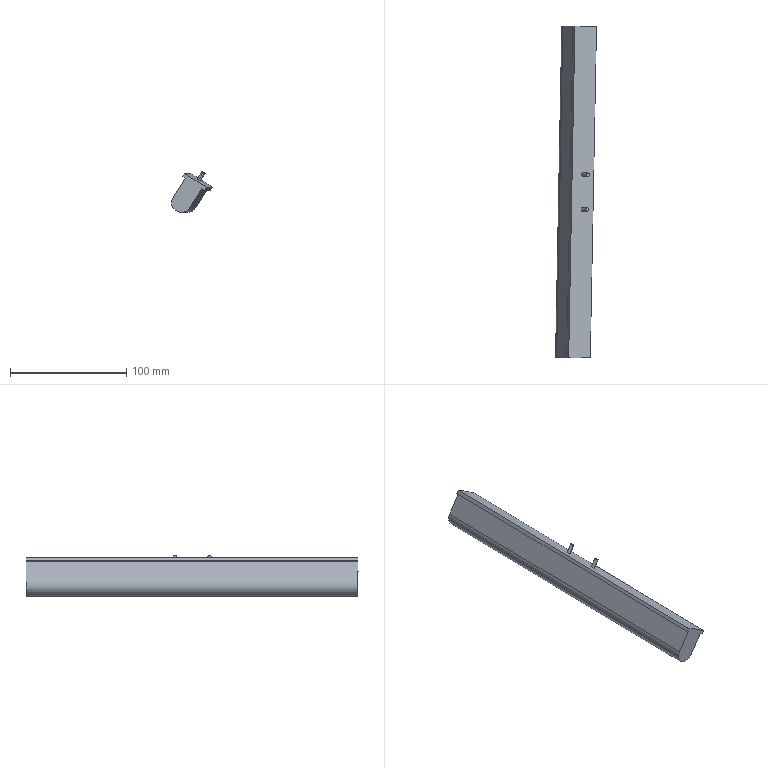Component | SolidWorks | LowerCameraLightSource-1 | 1 solid | 16 faces | box 35.21 x 285.51 x 35.02 mm | volume 145745 mm3 | plane 11 | cylinder 5 | commonest cylinder face diameters 3 x4 17 x1 | material PP Copolymer
build123d program:
from build123d import *

# Parameters (mm, degrees)
BOSS_EXTRUDE1_DEPTH = 142.5
SKETCH2_R           = 1.5
BOSS_EXTRUDE2_DEPTH = 8


with BuildPart() as part:
    # Sketch1 → Boss-Extrude1 (new, symmetric)
    with BuildSketch(Plane.XY):
        with BuildLine():
            Line((-8.5, 0), (-8.5, -19.5))
            Line((-8.5, -19.5), (-11, -19.5))
            Line((-11, -19.5), (-11, -22.5))
            Line((-11, -22.5), (11, -22.5))
            Line((11, -22.5), (11, -19.5))
            Line((11, -19.5), (8.5, -19.5))
            Line((8.5, -19.5), (8.5, 0))
            ThreePointArc((8.5, 0), (0, 8.5), (-8.5, 0))
        make_face()
    extrude(amount=BOSS_EXTRUDE1_DEPTH, both=True)

    # Sketch2 → Boss-Extrude2 (add)
    with BuildSketch(Plane.XZ.offset(22.5)):
        with Locations(Location((0, -15, 0), (0, 0, 90))):
            Circle(SKETCH2_R)
        with Locations(Location((0, 15, 0), (0, 0, 90))):
            Circle(SKETCH2_R)
    extrude(amount=BOSS_EXTRUDE2_DEPTH)


solid = part.part

# Placed as in the assembly
solid = solid.moved(Location((590.931, 385.027, 902.845), (90, -1.073, 147.47)))
STEP:
#1=CARTESIAN_POINT('',(23.901,14.615,36.557));
#2=VERTEX_POINT('',#1);
#3=CARTESIAN_POINT('',(23.898,14.497,36.557));
#4=VERTEX_POINT('',#3);
#5=CARTESIAN_POINT('',(23.9,14.556,36.557));
#6=DIRECTION('',(0.5377,-0.01007,0.8431));
#7=DIRECTION('',(-0.01873,-0.9998,0.));
#8=AXIS2_PLACEMENT_3D('',#5,#6,#7);
#9=CIRCLE('',#8,0.05906);
#10=EDGE_CURVE('',#2,#4,#9,.T.);
#11=ORIENTED_EDGE('',*,*,#10,.F.);
#12=CARTESIAN_POINT('',(23.731,14.618,36.292));
#13=VERTEX_POINT('',#12);
#14=CARTESIAN_POINT('',(23.901,14.615,36.557));
#15=DIRECTION('',(-0.5377,0.01007,-0.8431));
#16=VECTOR('',#15,39.37);
#17=LINE('',#14,#16);
#18=EDGE_CURVE('',#2,#13,#17,.T.);
#19=ORIENTED_EDGE('',*,*,#18,.T.);
#20=CARTESIAN_POINT('',(23.729,14.5,36.292));
#21=VERTEX_POINT('',#20);
#22=CARTESIAN_POINT('',(23.73,14.559,36.292));
#23=DIRECTION('',(0.5377,-0.01007,0.8431));
#24=DIRECTION('',(-0.01873,-0.9998,0.));
#25=AXIS2_PLACEMENT_3D('',#22,#23,#24);
#26=CIRCLE('',#25,0.05906);
#27=EDGE_CURVE('',#13,#21,#26,.T.);
#28=ORIENTED_EDGE('',*,*,#27,.T.);
#29=CARTESIAN_POINT('',(23.898,14.497,36.557));
#30=DIRECTION('',(-0.5377,0.01007,-0.8431));
#31=VECTOR('',#30,39.37);
#32=LINE('',#29,#31);
#33=EDGE_CURVE('',#4,#21,#32,.T.);
#34=ORIENTED_EDGE('',*,*,#33,.F.);
#35=EDGE_LOOP('',(#11,#19,#28,#34));
#36=FACE_OUTER_BOUND('',#35,.T.);
#37=CARTESIAN_POINT('',(23.9,14.556,36.557));
#38=DIRECTION('',(-0.5377,0.01007,-0.8431));
#39=DIRECTION('',(-0.01873,-0.9998,0.));
#40=AXIS2_PLACEMENT_3D('',#37,#38,#39);
#41=CYLINDRICAL_SURFACE('',#40,0.05906);
#42=ADVANCED_FACE('',(#36),#41,.T.);
#43=CARTESIAN_POINT('',(23.923,15.796,36.557));
#44=VERTEX_POINT('',#43);
#45=CARTESIAN_POINT('',(23.921,15.678,36.557));
#46=VERTEX_POINT('',#45);
#47=CARTESIAN_POINT('',(23.922,15.737,36.557));
#48=DIRECTION('',(0.5377,-0.01007,0.8431));
#49=DIRECTION('',(0.01873,0.9998,0.));
#50=AXIS2_PLACEMENT_3D('',#47,#48,#49);
#51=CIRCLE('',#50,0.05906);
#52=EDGE_CURVE('',#44,#46,#51,.T.);
#53=ORIENTED_EDGE('',*,*,#52,.F.);
#54=CARTESIAN_POINT('',(23.753,15.799,36.292));
#55=VERTEX_POINT('',#54);
#56=CARTESIAN_POINT('',(23.923,15.796,36.557));
#57=DIRECTION('',(-0.5377,0.01007,-0.8431));
#58=VECTOR('',#57,39.37);
#59=LINE('',#56,#58);
#60=EDGE_CURVE('',#44,#55,#59,.T.);
#61=ORIENTED_EDGE('',*,*,#60,.T.);
#62=CARTESIAN_POINT('',(23.751,15.681,36.292));
#63=VERTEX_POINT('',#62);
#64=CARTESIAN_POINT('',(23.752,15.74,36.292));
#65=DIRECTION('',(0.5377,-0.01007,0.8431));
#66=DIRECTION('',(-0.01873,-0.9998,0.));
#67=AXIS2_PLACEMENT_3D('',#64,#65,#66);
#68=CIRCLE('',#67,0.05906);
#69=EDGE_CURVE('',#55,#63,#68,.T.);
#70=ORIENTED_EDGE('',*,*,#69,.T.);
#71=CARTESIAN_POINT('',(23.921,15.678,36.557));
#72=DIRECTION('',(-0.5377,0.01007,-0.8431));
#73=VECTOR('',#72,39.37);
#74=LINE('',#71,#73);
#75=EDGE_CURVE('',#46,#63,#74,.T.);
#76=ORIENTED_EDGE('',*,*,#75,.F.);
#77=EDGE_LOOP('',(#53,#61,#70,#76));
#78=FACE_OUTER_BOUND('',#77,.T.);
#79=CARTESIAN_POINT('',(23.922,15.737,36.557));
#80=DIRECTION('',(-0.5377,0.01007,-0.8431));
#81=DIRECTION('',(-0.01873,-0.9998,0.));
#82=AXIS2_PLACEMENT_3D('',#79,#80,#81);
#83=CYLINDRICAL_SURFACE('',#82,0.05906);
#84=ADVANCED_FACE('',(#78),#83,.T.);
#85=CARTESIAN_POINT('',(23.088,20.773,35.725));
#86=VERTEX_POINT('',#85);
#87=CARTESIAN_POINT('',(23.652,20.763,35.365));
#88=VERTEX_POINT('',#87);
#89=CARTESIAN_POINT('',(23.37,20.768,35.545));
#90=DIRECTION('',(-0.01873,-0.9998,0.));
#91=DIRECTION('',(-0.843,0.01579,0.5377));
#92=AXIS2_PLACEMENT_3D('',#89,#90,#91);
#93=CIRCLE('',#92,0.3346);
#94=EDGE_CURVE('',#86,#88,#93,.T.);
#95=ORIENTED_EDGE('',*,*,#94,.T.);
#96=CARTESIAN_POINT('',(23.442,9.544,35.365));
#97=VERTEX_POINT('',#96);
#98=CARTESIAN_POINT('',(23.442,9.544,35.365));
#99=DIRECTION('',(0.01873,0.9998,-0.));
#100=VECTOR('',#99,39.37);
#101=LINE('',#98,#100);
#102=EDGE_CURVE('',#97,#88,#101,.T.);
#103=ORIENTED_EDGE('',*,*,#102,.F.);
#104=CARTESIAN_POINT('',(22.878,9.555,35.725));
#105=VERTEX_POINT('',#104);
#106=CARTESIAN_POINT('',(23.16,9.549,35.545));
#107=DIRECTION('',(-0.01873,-0.9998,0.));
#108=DIRECTION('',(-0.843,0.01579,0.5377));
#109=AXIS2_PLACEMENT_3D('',#106,#107,#108);
#110=CIRCLE('',#109,0.3346);
#111=EDGE_CURVE('',#105,#97,#110,.T.);
#112=ORIENTED_EDGE('',*,*,#111,.F.);
#113=CARTESIAN_POINT('',(22.878,9.555,35.725));
#114=DIRECTION('',(0.01873,0.9998,-0.));
#115=VECTOR('',#114,39.37);
#116=LINE('',#113,#115);
#117=EDGE_CURVE('',#105,#86,#116,.T.);
#118=ORIENTED_EDGE('',*,*,#117,.T.);
#119=EDGE_LOOP('',(#95,#103,#112,#118));
#120=FACE_OUTER_BOUND('',#119,.T.);
#121=CARTESIAN_POINT('',(23.16,9.549,35.545));
#122=DIRECTION('',(0.01873,0.9998,-0.));
#123=DIRECTION('',(0.843,-0.01579,-0.5377));
#124=AXIS2_PLACEMENT_3D('',#121,#122,#123);
#125=CYLINDRICAL_SURFACE('',#124,0.3346);
#126=ADVANCED_FACE('',(#120),#125,.T.);
#127=CARTESIAN_POINT('',(24.065,20.755,36.012));
#128=VERTEX_POINT('',#127);
#129=CARTESIAN_POINT('',(23.652,20.763,35.365));
#130=DIRECTION('',(0.5377,-0.01007,0.8431));
#131=VECTOR('',#130,39.37);
#132=LINE('',#129,#131);
#133=EDGE_CURVE('',#88,#128,#132,.T.);
#134=ORIENTED_EDGE('',*,*,#133,.T.);
#135=CARTESIAN_POINT('',(23.855,9.536,36.012));
#136=VERTEX_POINT('',#135);
#137=CARTESIAN_POINT('',(23.855,9.536,36.012));
#138=DIRECTION('',(0.01873,0.9998,-0.));
#139=VECTOR('',#138,39.37);
#140=LINE('',#137,#139);
#141=EDGE_CURVE('',#136,#128,#140,.T.);
#142=ORIENTED_EDGE('',*,*,#141,.F.);
#143=CARTESIAN_POINT('',(23.442,9.544,35.365));
#144=DIRECTION('',(0.5377,-0.01007,0.8431));
#145=VECTOR('',#144,39.37);
#146=LINE('',#143,#145);
#147=EDGE_CURVE('',#97,#136,#146,.T.);
#148=ORIENTED_EDGE('',*,*,#147,.F.);
#149=ORIENTED_EDGE('',*,*,#102,.T.);
#150=EDGE_LOOP('',(#134,#142,#148,#149));
#151=FACE_OUTER_BOUND('',#150,.T.);
#152=CARTESIAN_POINT('',(23.442,9.544,35.365));
#153=DIRECTION('',(-0.843,0.01579,0.5377));
#154=DIRECTION('',(0.01873,0.9998,-0.));
#155=AXIS2_PLACEMENT_3D('',#152,#153,#154);
#156=PLANE('',#155);
#157=ADVANCED_FACE('',(#151),#156,.F.);
#158=CARTESIAN_POINT('',(24.148,20.753,35.959));
#159=VERTEX_POINT('',#158);
#160=CARTESIAN_POINT('',(24.065,20.755,36.012));
#161=DIRECTION('',(0.843,-0.01579,-0.5377));
#162=VECTOR('',#161,39.37);
#163=LINE('',#160,#162);
#164=EDGE_CURVE('',#128,#159,#163,.T.);
#165=ORIENTED_EDGE('',*,*,#164,.T.);
#166=CARTESIAN_POINT('',(23.938,9.535,35.959));
#167=VERTEX_POINT('',#166);
#168=CARTESIAN_POINT('',(23.938,9.535,35.959));
#169=DIRECTION('',(0.01873,0.9998,-0.));
#170=VECTOR('',#169,39.37);
#171=LINE('',#168,#170);
#172=EDGE_CURVE('',#167,#159,#171,.T.);
#173=ORIENTED_EDGE('',*,*,#172,.F.);
#174=CARTESIAN_POINT('',(23.855,9.536,36.012));
#175=DIRECTION('',(0.843,-0.01579,-0.5377));
#176=VECTOR('',#175,39.37);
#177=LINE('',#174,#176);
#178=EDGE_CURVE('',#136,#167,#177,.T.);
#179=ORIENTED_EDGE('',*,*,#178,.F.);
#180=ORIENTED_EDGE('',*,*,#141,.T.);
#181=EDGE_LOOP('',(#165,#173,#179,#180));
#182=FACE_OUTER_BOUND('',#181,.T.);
#183=CARTESIAN_POINT('',(23.855,9.536,36.012));
#184=DIRECTION('',(0.5377,-0.01007,0.8431));
#185=DIRECTION('',(-0.843,0.01579,0.5377));
#186=AXIS2_PLACEMENT_3D('',#183,#184,#185);
#187=PLANE('',#186);
#188=ADVANCED_FACE('',(#182),#187,.F.);
#189=CARTESIAN_POINT('',(24.211,20.752,36.059));
#190=VERTEX_POINT('',#189);
#191=CARTESIAN_POINT('',(24.148,20.753,35.959));
#192=DIRECTION('',(0.5377,-0.01007,0.8431));
#193=VECTOR('',#192,39.37);
#194=LINE('',#191,#193);
#195=EDGE_CURVE('',#159,#190,#194,.T.);
#196=ORIENTED_EDGE('',*,*,#195,.T.);
#197=CARTESIAN_POINT('',(24.001,9.534,36.059));
#198=VERTEX_POINT('',#197);
#199=CARTESIAN_POINT('',(24.001,9.534,36.059));
#200=DIRECTION('',(0.01873,0.9998,-0.));
#201=VECTOR('',#200,39.37);
#202=LINE('',#199,#201);
#203=EDGE_CURVE('',#198,#190,#202,.T.);
#204=ORIENTED_EDGE('',*,*,#203,.F.);
#205=CARTESIAN_POINT('',(23.938,9.535,35.959));
#206=DIRECTION('',(0.5377,-0.01007,0.8431));
#207=VECTOR('',#206,39.37);
#208=LINE('',#205,#207);
#209=EDGE_CURVE('',#167,#198,#208,.T.);
#210=ORIENTED_EDGE('',*,*,#209,.F.);
#211=ORIENTED_EDGE('',*,*,#172,.T.);
#212=EDGE_LOOP('',(#196,#204,#210,#211));
#213=FACE_OUTER_BOUND('',#212,.T.);
#214=CARTESIAN_POINT('',(23.938,9.535,35.959));
#215=DIRECTION('',(-0.843,0.01579,0.5377));
#216=DIRECTION('',(0.01873,0.9998,-0.));
#217=AXIS2_PLACEMENT_3D('',#214,#215,#216);
#218=PLANE('',#217);
#219=ADVANCED_FACE('',(#213),#218,.F.);
#220=CARTESIAN_POINT('',(23.73,14.559,36.292));
#221=DIRECTION('',(0.5377,-0.01007,0.8431));
#222=DIRECTION('',(-0.01873,-0.9998,0.));
#223=AXIS2_PLACEMENT_3D('',#220,#221,#222);
#224=CIRCLE('',#223,0.05906);
#225=EDGE_CURVE('',#21,#13,#224,.T.);
#226=ORIENTED_EDGE('',*,*,#225,.F.);
#227=ORIENTED_EDGE('',*,*,#27,.F.);
#228=EDGE_LOOP('',(#226,#227));
#229=FACE_BOUND('',#228,.T.);
#230=CARTESIAN_POINT('',(23.752,15.74,36.292));
#231=DIRECTION('',(0.5377,-0.01007,0.8431));
#232=DIRECTION('',(-0.01873,-0.9998,0.));
#233=AXIS2_PLACEMENT_3D('',#230,#231,#232);
#234=CIRCLE('',#233,0.05906);
#235=EDGE_CURVE('',#63,#55,#234,.T.);
#236=ORIENTED_EDGE('',*,*,#235,.F.);
#237=ORIENTED_EDGE('',*,*,#69,.F.);
#238=EDGE_LOOP('',(#236,#237));
#239=FACE_BOUND('',#238,.T.);
#240=CARTESIAN_POINT('',(23.481,20.766,36.525));
#241=VERTEX_POINT('',#240);
#242=CARTESIAN_POINT('',(24.211,20.752,36.059));
#243=DIRECTION('',(-0.843,0.01579,0.5377));
#244=VECTOR('',#243,39.37);
#245=LINE('',#242,#244);
#246=EDGE_CURVE('',#190,#241,#245,.T.);
#247=ORIENTED_EDGE('',*,*,#246,.T.);
#248=CARTESIAN_POINT('',(23.271,9.547,36.525));
#249=VERTEX_POINT('',#248);
#250=CARTESIAN_POINT('',(23.271,9.547,36.525));
#251=DIRECTION('',(0.01873,0.9998,-0.));
#252=VECTOR('',#251,39.37);
#253=LINE('',#250,#252);
#254=EDGE_CURVE('',#249,#241,#253,.T.);
#255=ORIENTED_EDGE('',*,*,#254,.F.);
#256=CARTESIAN_POINT('',(24.001,9.534,36.059));
#257=DIRECTION('',(-0.843,0.01579,0.5377));
#258=VECTOR('',#257,39.37);
#259=LINE('',#256,#258);
#260=EDGE_CURVE('',#198,#249,#259,.T.);
#261=ORIENTED_EDGE('',*,*,#260,.F.);
#262=ORIENTED_EDGE('',*,*,#203,.T.);
#263=EDGE_LOOP('',(#247,#255,#261,#262));
#264=FACE_OUTER_BOUND('',#263,.T.);
#265=CARTESIAN_POINT('',(24.001,9.534,36.059));
#266=DIRECTION('',(-0.5377,0.01007,-0.8431));
#267=DIRECTION('',(-0.01873,-0.9998,0.));
#268=AXIS2_PLACEMENT_3D('',#265,#266,#267);
#269=PLANE('',#268);
#270=ADVANCED_FACE('',(#229,#239,#264),#269,.F.);
#271=CARTESIAN_POINT('',(23.418,20.767,36.425));
#272=VERTEX_POINT('',#271);
#273=CARTESIAN_POINT('',(23.418,20.767,36.425));
#274=DIRECTION('',(-0.5377,0.01007,-0.8431));
#275=VECTOR('',#274,39.37);
#276=LINE('',#273,#275);
#277=EDGE_CURVE('',#241,#272,#276,.T.);
#278=ORIENTED_EDGE('',*,*,#277,.T.);
#279=CARTESIAN_POINT('',(23.208,9.548,36.425));
#280=VERTEX_POINT('',#279);
#281=CARTESIAN_POINT('',(23.208,9.548,36.425));
#282=DIRECTION('',(0.01873,0.9998,-0.));
#283=VECTOR('',#282,39.37);
#284=LINE('',#281,#283);
#285=EDGE_CURVE('',#280,#272,#284,.T.);
#286=ORIENTED_EDGE('',*,*,#285,.F.);
#287=CARTESIAN_POINT('',(23.208,9.548,36.425));
#288=DIRECTION('',(-0.5377,0.01007,-0.8431));
#289=VECTOR('',#288,39.37);
#290=LINE('',#287,#289);
#291=EDGE_CURVE('',#249,#280,#290,.T.);
#292=ORIENTED_EDGE('',*,*,#291,.F.);
#293=ORIENTED_EDGE('',*,*,#254,.T.);
#294=EDGE_LOOP('',(#278,#286,#292,#293));
#295=FACE_OUTER_BOUND('',#294,.T.);
#296=CARTESIAN_POINT('',(23.208,9.548,36.425));
#297=DIRECTION('',(0.843,-0.01579,-0.5377));
#298=DIRECTION('',(-0.01873,-0.9998,0.));
#299=AXIS2_PLACEMENT_3D('',#296,#297,#298);
#300=PLANE('',#299);
#301=ADVANCED_FACE('',(#295),#300,.F.);
#302=CARTESIAN_POINT('',(23.501,20.765,36.372));
#303=VERTEX_POINT('',#302);
#304=CARTESIAN_POINT('',(23.501,20.765,36.372));
#305=DIRECTION('',(0.843,-0.01579,-0.5377));
#306=VECTOR('',#305,39.37);
#307=LINE('',#304,#306);
#308=EDGE_CURVE('',#272,#303,#307,.T.);
#309=ORIENTED_EDGE('',*,*,#308,.T.);
#310=CARTESIAN_POINT('',(23.291,9.547,36.372));
#311=VERTEX_POINT('',#310);
#312=CARTESIAN_POINT('',(23.291,9.547,36.372));
#313=DIRECTION('',(0.01873,0.9998,-0.));
#314=VECTOR('',#313,39.37);
#315=LINE('',#312,#314);
#316=EDGE_CURVE('',#311,#303,#315,.T.);
#317=ORIENTED_EDGE('',*,*,#316,.F.);
#318=CARTESIAN_POINT('',(23.291,9.547,36.372));
#319=DIRECTION('',(0.843,-0.01579,-0.5377));
#320=VECTOR('',#319,39.37);
#321=LINE('',#318,#320);
#322=EDGE_CURVE('',#280,#311,#321,.T.);
#323=ORIENTED_EDGE('',*,*,#322,.F.);
#324=ORIENTED_EDGE('',*,*,#285,.T.);
#325=EDGE_LOOP('',(#309,#317,#323,#324));
#326=FACE_OUTER_BOUND('',#325,.T.);
#327=CARTESIAN_POINT('',(23.291,9.547,36.372));
#328=DIRECTION('',(0.5377,-0.01007,0.8431));
#329=DIRECTION('',(-0.843,0.01579,0.5377));
#330=AXIS2_PLACEMENT_3D('',#327,#328,#329);
#331=PLANE('',#330);
#332=ADVANCED_FACE('',(#326),#331,.F.);
#333=CARTESIAN_POINT('',(23.088,20.773,35.725));
#334=DIRECTION('',(-0.5377,0.01007,-0.8431));
#335=VECTOR('',#334,39.37);
#336=LINE('',#333,#335);
#337=EDGE_CURVE('',#303,#86,#336,.T.);
#338=ORIENTED_EDGE('',*,*,#337,.T.);
#339=ORIENTED_EDGE('',*,*,#117,.F.);
#340=CARTESIAN_POINT('',(22.878,9.555,35.725));
#341=DIRECTION('',(-0.5377,0.01007,-0.8431));
#342=VECTOR('',#341,39.37);
#343=LINE('',#340,#342);
#344=EDGE_CURVE('',#311,#105,#343,.T.);
#345=ORIENTED_EDGE('',*,*,#344,.F.);
#346=ORIENTED_EDGE('',*,*,#316,.T.);
#347=EDGE_LOOP('',(#338,#339,#345,#346));
#348=FACE_OUTER_BOUND('',#347,.T.);
#349=CARTESIAN_POINT('',(22.878,9.555,35.725));
#350=DIRECTION('',(0.843,-0.01579,-0.5377));
#351=DIRECTION('',(-0.01873,-0.9998,0.));
#352=AXIS2_PLACEMENT_3D('',#349,#350,#351);
#353=PLANE('',#352);
#354=ADVANCED_FACE('',(#348),#353,.F.);
#355=ORIENTED_EDGE('',*,*,#111,.T.);
#356=ORIENTED_EDGE('',*,*,#147,.T.);
#357=ORIENTED_EDGE('',*,*,#178,.T.);
#358=ORIENTED_EDGE('',*,*,#209,.T.);
#359=ORIENTED_EDGE('',*,*,#260,.T.);
#360=ORIENTED_EDGE('',*,*,#291,.T.);
#361=ORIENTED_EDGE('',*,*,#322,.T.);
#362=ORIENTED_EDGE('',*,*,#344,.T.);
#363=EDGE_LOOP('',(#355,#356,#357,#358,#359,#360,#361,#362));
#364=FACE_OUTER_BOUND('',#363,.T.);
#365=CARTESIAN_POINT('',(23.16,9.549,35.545));
#366=DIRECTION('',(-0.01873,-0.9998,0.));
#367=DIRECTION('',(-0.843,0.01579,0.5377));
#368=AXIS2_PLACEMENT_3D('',#365,#366,#367);
#369=PLANE('',#368);
#370=ADVANCED_FACE('',(#364),#369,.T.);
#371=ORIENTED_EDGE('',*,*,#94,.F.);
#372=ORIENTED_EDGE('',*,*,#337,.F.);
#373=ORIENTED_EDGE('',*,*,#308,.F.);
#374=ORIENTED_EDGE('',*,*,#277,.F.);
#375=ORIENTED_EDGE('',*,*,#246,.F.);
#376=ORIENTED_EDGE('',*,*,#195,.F.);
#377=ORIENTED_EDGE('',*,*,#164,.F.);
#378=ORIENTED_EDGE('',*,*,#133,.F.);
#379=EDGE_LOOP('',(#371,#372,#373,#374,#375,#376,#377,#378));
#380=FACE_OUTER_BOUND('',#379,.T.);
#381=CARTESIAN_POINT('',(23.37,20.768,35.545));
#382=DIRECTION('',(-0.01873,-0.9998,0.));
#383=DIRECTION('',(-0.843,0.01579,0.5377));
#384=AXIS2_PLACEMENT_3D('',#381,#382,#383);
#385=PLANE('',#384);
#386=ADVANCED_FACE('',(#380),#385,.F.);
#387=ORIENTED_EDGE('',*,*,#60,.F.);
#388=CARTESIAN_POINT('',(23.922,15.737,36.557));
#389=DIRECTION('',(0.5377,-0.01007,0.8431));
#390=DIRECTION('',(0.01873,0.9998,0.));
#391=AXIS2_PLACEMENT_3D('',#388,#389,#390);
#392=CIRCLE('',#391,0.05906);
#393=EDGE_CURVE('',#46,#44,#392,.T.);
#394=ORIENTED_EDGE('',*,*,#393,.F.);
#395=ORIENTED_EDGE('',*,*,#75,.T.);
#396=ORIENTED_EDGE('',*,*,#235,.T.);
#397=EDGE_LOOP('',(#387,#394,#395,#396));
#398=FACE_OUTER_BOUND('',#397,.T.);
#399=CARTESIAN_POINT('',(23.922,15.737,36.557));
#400=DIRECTION('',(-0.5377,0.01007,-0.8431));
#401=DIRECTION('',(-0.01873,-0.9998,0.));
#402=AXIS2_PLACEMENT_3D('',#399,#400,#401);
#403=CYLINDRICAL_SURFACE('',#402,0.05906);
#404=ADVANCED_FACE('',(#398),#403,.T.);
#405=ORIENTED_EDGE('',*,*,#393,.T.);
#406=ORIENTED_EDGE('',*,*,#52,.T.);
#407=EDGE_LOOP('',(#405,#406));
#408=FACE_OUTER_BOUND('',#407,.T.);
#409=CARTESIAN_POINT('',(23.922,15.737,36.557));
#410=DIRECTION('',(0.5377,-0.01007,0.8431));
#411=DIRECTION('',(0.01873,0.9998,-0.));
#412=AXIS2_PLACEMENT_3D('',#409,#410,#411);
#413=PLANE('',#412);
#414=ADVANCED_FACE('',(#408),#413,.T.);
#415=ORIENTED_EDGE('',*,*,#18,.F.);
#416=CARTESIAN_POINT('',(23.9,14.556,36.557));
#417=DIRECTION('',(0.5377,-0.01007,0.8431));
#418=DIRECTION('',(-0.01873,-0.9998,0.));
#419=AXIS2_PLACEMENT_3D('',#416,#417,#418);
#420=CIRCLE('',#419,0.05906);
#421=EDGE_CURVE('',#4,#2,#420,.T.);
#422=ORIENTED_EDGE('',*,*,#421,.F.);
#423=ORIENTED_EDGE('',*,*,#33,.T.);
#424=ORIENTED_EDGE('',*,*,#225,.T.);
#425=EDGE_LOOP('',(#415,#422,#423,#424));
#426=FACE_OUTER_BOUND('',#425,.T.);
#427=CARTESIAN_POINT('',(23.9,14.556,36.557));
#428=DIRECTION('',(-0.5377,0.01007,-0.8431));
#429=DIRECTION('',(-0.01873,-0.9998,0.));
#430=AXIS2_PLACEMENT_3D('',#427,#428,#429);
#431=CYLINDRICAL_SURFACE('',#430,0.05906);
#432=ADVANCED_FACE('',(#426),#431,.T.);
#433=ORIENTED_EDGE('',*,*,#421,.T.);
#434=ORIENTED_EDGE('',*,*,#10,.T.);
#435=EDGE_LOOP('',(#433,#434));
#436=FACE_OUTER_BOUND('',#435,.T.);
#437=CARTESIAN_POINT('',(23.9,14.556,36.557));
#438=DIRECTION('',(-0.5377,0.01007,-0.8431));
#439=DIRECTION('',(-0.01873,-0.9998,0.));
#440=AXIS2_PLACEMENT_3D('',#437,#438,#439);
#441=PLANE('',#440);
#442=ADVANCED_FACE('',(#436),#441,.F.);
#443=CLOSED_SHELL('',(#42,#84,#126,#157,#188,#219,#270,#301,#332,#354,#370,#386,#404,#414,#432,#442));
#444=MANIFOLD_SOLID_BREP('',#443);
#445=CARTESIAN_POINT('',(0.,0.,0.));
#446=DIRECTION('',(0.,0.,1.));
#447=DIRECTION('',(1.,0.,0.));
#448=AXIS2_PLACEMENT_3D('',#445,#446,#447);
#449=(LENGTH_UNIT()NAMED_UNIT(*)SI_UNIT($,.METRE.));
#450=LENGTH_MEASURE_WITH_UNIT(LENGTH_MEASURE(0.0254),#449);
#451=DIMENSIONAL_EXPONENTS(1.,0.,0.,0.,0.,0.,0.);
#452=(CONVERSION_BASED_UNIT('',#450)LENGTH_UNIT()NAMED_UNIT(#451));
#453=UNCERTAINTY_MEASURE_WITH_UNIT(LENGTH_MEASURE(0.00001),#452,'','');
#454=(NAMED_UNIT(*)PLANE_ANGLE_UNIT()SI_UNIT($,.RADIAN.));
#455=(NAMED_UNIT(*)SI_UNIT($,.STERADIAN.)SOLID_ANGLE_UNIT());
#456=(GEOMETRIC_REPRESENTATION_CONTEXT(3)GLOBAL_UNCERTAINTY_ASSIGNED_CONTEXT((#453))GLOBAL_UNIT_ASSIGNED_CONTEXT((#452,#454,#455))REPRESENTATION_CONTEXT('',''));
#457=ADVANCED_BREP_SHAPE_REPRESENTATION('',(#444,#448),#456);
#458=COLOUR_RGB('',0.7922,0.8196,0.9333);
#459=FILL_AREA_STYLE_COLOUR('',#458);
#460=FILL_AREA_STYLE('',(#459));
#461=SURFACE_STYLE_FILL_AREA(#460);
#462=SURFACE_SIDE_STYLE('',(#461));
#463=SURFACE_STYLE_USAGE(.BOTH.,#462);
#464=PRESENTATION_STYLE_ASSIGNMENT((#463));
#465=STYLED_ITEM('',(#464),#444);
#466=PRESENTATION_LAYER_ASSIGNMENT('','',(#465));
#467=(LENGTH_UNIT()NAMED_UNIT(*)SI_UNIT($,.METRE.));
#468=LENGTH_MEASURE_WITH_UNIT(LENGTH_MEASURE(0.0254),#467);
#469=DIMENSIONAL_EXPONENTS(1.,0.,0.,0.,0.,0.,0.);
#470=(CONVERSION_BASED_UNIT('',#468)LENGTH_UNIT()NAMED_UNIT(#469));
#471=UNCERTAINTY_MEASURE_WITH_UNIT(LENGTH_MEASURE(0.00001),#470,'','');
#472=(NAMED_UNIT(*)PLANE_ANGLE_UNIT()SI_UNIT($,.RADIAN.));
#473=(NAMED_UNIT(*)SI_UNIT($,.STERADIAN.)SOLID_ANGLE_UNIT());
#474=(GEOMETRIC_REPRESENTATION_CONTEXT(3)GLOBAL_UNCERTAINTY_ASSIGNED_CONTEXT((#471))GLOBAL_UNIT_ASSIGNED_CONTEXT((#470,#472,#473))REPRESENTATION_CONTEXT('',''));
#475=MECHANICAL_DESIGN_GEOMETRIC_PRESENTATION_REPRESENTATION('',(#465),#474);